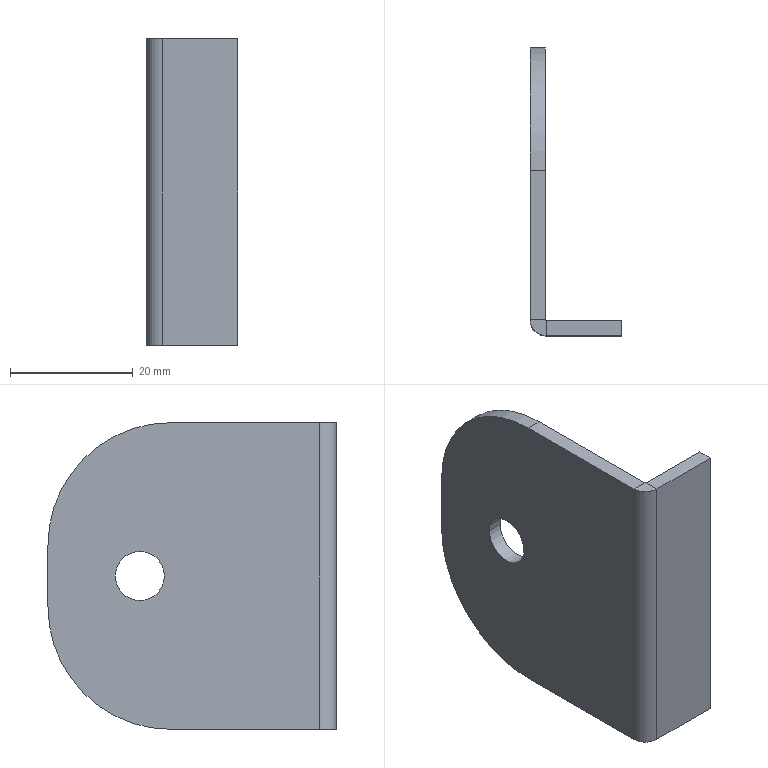Component | SolidWorks | FrontDoorAssembly-1_FrontDoorWelding-1_GasSpringSupportPG50-02-104-1 | 1 solid | 18 faces | box 15 x 47 x 50 mm | volume 6808 mm3 | plane 12 | cylinder 6 | commonest cylinder face diameters 8 x2 40 x2 5.3 x1 0.3 x1 | material AISI 1045 Steel, cold drawn
STEP:
#1=COLOUR_RGB('',0.7922,0.8196,0.9333);
#2=FILL_AREA_STYLE_COLOUR('',#1);
#3=FILL_AREA_STYLE('',(#2));
#4=SURFACE_STYLE_FILL_AREA(#3);
#5=SURFACE_SIDE_STYLE('',(#4));
#6=SURFACE_STYLE_USAGE(.BOTH.,#5);
#7=PRESENTATION_STYLE_ASSIGNMENT((#6));
#8=CARTESIAN_POINT('',(34.914,-9.992,-0.3876));
#9=VERTEX_POINT('',#8);
#10=CARTESIAN_POINT('',(34.914,-9.677,-0.3876));
#11=VERTEX_POINT('',#10);
#12=CARTESIAN_POINT('',(34.914,-9.835,-0.3876));
#13=DIRECTION('',(-1.,-0.,0.));
#14=DIRECTION('',(0.,1.,0.));
#15=AXIS2_PLACEMENT_3D('',#12,#13,#14);
#16=CIRCLE('',#15,0.1575);
#17=EDGE_CURVE('',#9,#11,#16,.T.);
#18=ORIENTED_EDGE('',*,*,#17,.F.);
#19=CARTESIAN_POINT('',(34.816,-9.992,-0.3876));
#20=VERTEX_POINT('',#19);
#21=CARTESIAN_POINT('',(34.914,-9.992,-0.3876));
#22=DIRECTION('',(-1.,-0.,0.));
#23=VECTOR('',#22,39.37);
#24=LINE('',#21,#23);
#25=EDGE_CURVE('',#9,#20,#24,.T.);
#26=ORIENTED_EDGE('',*,*,#25,.T.);
#27=CARTESIAN_POINT('',(34.816,-9.677,-0.3876));
#28=VERTEX_POINT('',#27);
#29=CARTESIAN_POINT('',(34.816,-9.835,-0.3876));
#30=DIRECTION('',(-1.,-0.,0.));
#31=DIRECTION('',(0.,1.,0.));
#32=AXIS2_PLACEMENT_3D('',#29,#30,#31);
#33=CIRCLE('',#32,0.1575);
#34=EDGE_CURVE('',#20,#28,#33,.T.);
#35=ORIENTED_EDGE('',*,*,#34,.T.);
#36=CARTESIAN_POINT('',(34.914,-9.677,-0.3876));
#37=DIRECTION('',(-1.,-0.,0.));
#38=VECTOR('',#37,39.37);
#39=LINE('',#36,#38);
#40=EDGE_CURVE('',#11,#28,#39,.T.);
#41=ORIENTED_EDGE('',*,*,#40,.F.);
#42=EDGE_LOOP('',(#18,#26,#35,#41));
#43=FACE_OUTER_BOUND('',#42,.T.);
#44=CARTESIAN_POINT('',(34.914,-9.835,-0.3876));
#45=DIRECTION('',(-1.,-0.,0.));
#46=DIRECTION('',(0.,1.,0.));
#47=AXIS2_PLACEMENT_3D('',#44,#45,#46);
#48=CYLINDRICAL_SURFACE('',#47,0.1575);
#49=ADVANCED_FACE('',(#43),#48,.F.);
#50=CARTESIAN_POINT('',(34.914,-10.031,-1.372));
#51=VERTEX_POINT('',#50);
#52=CARTESIAN_POINT('',(34.914,-10.99,-1.372));
#53=VERTEX_POINT('',#52);
#54=CARTESIAN_POINT('',(34.914,-10.031,-1.372));
#55=DIRECTION('',(0.,-1.,-0.));
#56=VECTOR('',#55,39.37);
#57=LINE('',#54,#56);
#58=EDGE_CURVE('',#51,#53,#57,.T.);
#59=ORIENTED_EDGE('',*,*,#58,.T.);
#60=CARTESIAN_POINT('',(34.816,-10.99,-1.372));
#61=VERTEX_POINT('',#60);
#62=CARTESIAN_POINT('',(34.914,-10.99,-1.372));
#63=DIRECTION('',(-1.,-0.,0.));
#64=VECTOR('',#63,39.37);
#65=LINE('',#62,#64);
#66=EDGE_CURVE('',#53,#61,#65,.T.);
#67=ORIENTED_EDGE('',*,*,#66,.T.);
#68=CARTESIAN_POINT('',(34.816,-10.031,-1.372));
#69=VERTEX_POINT('',#68);
#70=CARTESIAN_POINT('',(34.816,-10.031,-1.372));
#71=DIRECTION('',(0.,-1.,-0.));
#72=VECTOR('',#71,39.37);
#73=LINE('',#70,#72);
#74=EDGE_CURVE('',#69,#61,#73,.T.);
#75=ORIENTED_EDGE('',*,*,#74,.F.);
#76=CARTESIAN_POINT('',(34.914,-10.031,-1.372));
#77=DIRECTION('',(-1.,-0.,0.));
#78=VECTOR('',#77,39.37);
#79=LINE('',#76,#78);
#80=EDGE_CURVE('',#51,#69,#79,.T.);
#81=ORIENTED_EDGE('',*,*,#80,.F.);
#82=EDGE_LOOP('',(#59,#67,#75,#81));
#83=FACE_OUTER_BOUND('',#82,.T.);
#84=CARTESIAN_POINT('',(34.914,-10.031,-1.372));
#85=DIRECTION('',(-0.,0.,-1.));
#86=DIRECTION('',(-1.,-0.,0.));
#87=AXIS2_PLACEMENT_3D('',#84,#85,#86);
#88=PLANE('',#87);
#89=ADVANCED_FACE('',(#83),#88,.T.);
#90=CARTESIAN_POINT('',(34.914,-9.835,-0.3876));
#91=DIRECTION('',(-1.,-0.,0.));
#92=DIRECTION('',(0.,1.,0.));
#93=AXIS2_PLACEMENT_3D('',#90,#91,#92);
#94=CIRCLE('',#93,0.1575);
#95=EDGE_CURVE('',#11,#9,#94,.T.);
#96=ORIENTED_EDGE('',*,*,#95,.T.);
#97=ORIENTED_EDGE('',*,*,#17,.T.);
#98=EDGE_LOOP('',(#96,#97));
#99=FACE_BOUND('',#98,.T.);
#100=CARTESIAN_POINT('',(34.914,-10.99,0.5966));
#101=VERTEX_POINT('',#100);
#102=CARTESIAN_POINT('',(34.914,-10.99,-1.372));
#103=DIRECTION('',(0.,-0.,1.));
#104=VECTOR('',#103,39.37);
#105=LINE('',#102,#104);
#106=EDGE_CURVE('',#53,#101,#105,.T.);
#107=ORIENTED_EDGE('',*,*,#106,.F.);
#108=ORIENTED_EDGE('',*,*,#58,.F.);
#109=CARTESIAN_POINT('',(34.914,-9.244,-0.5845));
#110=VERTEX_POINT('',#109);
#111=CARTESIAN_POINT('',(34.914,-10.031,-0.5845));
#112=DIRECTION('',(-1.,-0.,0.));
#113=DIRECTION('',(-0.,1.,0.));
#114=AXIS2_PLACEMENT_3D('',#111,#112,#113);
#115=CIRCLE('',#114,0.7874);
#116=EDGE_CURVE('',#110,#51,#115,.T.);
#117=ORIENTED_EDGE('',*,*,#116,.F.);
#118=CARTESIAN_POINT('',(34.914,-9.244,-0.1908));
#119=VERTEX_POINT('',#118);
#120=CARTESIAN_POINT('',(34.914,-9.244,-0.1908));
#121=DIRECTION('',(-0.,0.,-1.));
#122=VECTOR('',#121,39.37);
#123=LINE('',#120,#122);
#124=EDGE_CURVE('',#119,#110,#123,.T.);
#125=ORIENTED_EDGE('',*,*,#124,.F.);
#126=CARTESIAN_POINT('',(34.914,-10.031,0.5966));
#127=VERTEX_POINT('',#126);
#128=CARTESIAN_POINT('',(34.914,-10.031,-0.1908));
#129=DIRECTION('',(-1.,-0.,0.));
#130=DIRECTION('',(-0.,1.,0.));
#131=AXIS2_PLACEMENT_3D('',#128,#129,#130);
#132=CIRCLE('',#131,0.7874);
#133=EDGE_CURVE('',#127,#119,#132,.T.);
#134=ORIENTED_EDGE('',*,*,#133,.F.);
#135=CARTESIAN_POINT('',(34.914,-11.094,0.5966));
#136=DIRECTION('',(-0.,1.,0.));
#137=VECTOR('',#136,39.37);
#138=LINE('',#135,#137);
#139=EDGE_CURVE('',#101,#127,#138,.T.);
#140=ORIENTED_EDGE('',*,*,#139,.F.);
#141=EDGE_LOOP('',(#107,#108,#117,#125,#134,#140));
#142=FACE_OUTER_BOUND('',#141,.T.);
#143=CARTESIAN_POINT('',(34.914,-10.031,-0.1908));
#144=DIRECTION('',(-1.,-0.,0.));
#145=DIRECTION('',(-0.,1.,0.));
#146=AXIS2_PLACEMENT_3D('',#143,#144,#145);
#147=PLANE('',#146);
#148=ADVANCED_FACE('',(#99,#142),#147,.F.);
#149=CARTESIAN_POINT('',(34.816,-9.835,-0.3876));
#150=DIRECTION('',(-1.,-0.,0.));
#151=DIRECTION('',(0.,1.,0.));
#152=AXIS2_PLACEMENT_3D('',#149,#150,#151);
#153=CIRCLE('',#152,0.1575);
#154=EDGE_CURVE('',#28,#20,#153,.T.);
#155=ORIENTED_EDGE('',*,*,#154,.F.);
#156=ORIENTED_EDGE('',*,*,#34,.F.);
#157=EDGE_LOOP('',(#155,#156));
#158=FACE_BOUND('',#157,.T.);
#159=ORIENTED_EDGE('',*,*,#74,.T.);
#160=CARTESIAN_POINT('',(34.816,-10.99,0.5966));
#161=VERTEX_POINT('',#160);
#162=CARTESIAN_POINT('',(34.816,-10.99,-1.372));
#163=DIRECTION('',(0.,-0.,1.));
#164=VECTOR('',#163,39.37);
#165=LINE('',#162,#164);
#166=EDGE_CURVE('',#61,#161,#165,.T.);
#167=ORIENTED_EDGE('',*,*,#166,.T.);
#168=CARTESIAN_POINT('',(34.816,-10.031,0.5966));
#169=VERTEX_POINT('',#168);
#170=CARTESIAN_POINT('',(34.816,-11.094,0.5966));
#171=DIRECTION('',(-0.,1.,0.));
#172=VECTOR('',#171,39.37);
#173=LINE('',#170,#172);
#174=EDGE_CURVE('',#161,#169,#173,.T.);
#175=ORIENTED_EDGE('',*,*,#174,.T.);
#176=CARTESIAN_POINT('',(34.816,-9.244,-0.1908));
#177=VERTEX_POINT('',#176);
#178=CARTESIAN_POINT('',(34.816,-10.031,-0.1908));
#179=DIRECTION('',(-1.,-0.,0.));
#180=DIRECTION('',(-0.,1.,0.));
#181=AXIS2_PLACEMENT_3D('',#178,#179,#180);
#182=CIRCLE('',#181,0.7874);
#183=EDGE_CURVE('',#169,#177,#182,.T.);
#184=ORIENTED_EDGE('',*,*,#183,.T.);
#185=CARTESIAN_POINT('',(34.816,-9.244,-0.5845));
#186=VERTEX_POINT('',#185);
#187=CARTESIAN_POINT('',(34.816,-9.244,-0.1908));
#188=DIRECTION('',(-0.,0.,-1.));
#189=VECTOR('',#188,39.37);
#190=LINE('',#187,#189);
#191=EDGE_CURVE('',#177,#186,#190,.T.);
#192=ORIENTED_EDGE('',*,*,#191,.T.);
#193=CARTESIAN_POINT('',(34.816,-10.031,-0.5845));
#194=DIRECTION('',(-1.,-0.,0.));
#195=DIRECTION('',(-0.,1.,0.));
#196=AXIS2_PLACEMENT_3D('',#193,#194,#195);
#197=CIRCLE('',#196,0.7874);
#198=EDGE_CURVE('',#186,#69,#197,.T.);
#199=ORIENTED_EDGE('',*,*,#198,.T.);
#200=EDGE_LOOP('',(#159,#167,#175,#184,#192,#199));
#201=FACE_OUTER_BOUND('',#200,.T.);
#202=CARTESIAN_POINT('',(34.816,-10.031,-0.1908));
#203=DIRECTION('',(-1.,-0.,0.));
#204=DIRECTION('',(-0.,1.,0.));
#205=AXIS2_PLACEMENT_3D('',#202,#203,#204);
#206=PLANE('',#205);
#207=ADVANCED_FACE('',(#158,#201),#206,.T.);
#208=ORIENTED_EDGE('',*,*,#198,.F.);
#209=CARTESIAN_POINT('',(34.914,-9.244,-0.5845));
#210=DIRECTION('',(-1.,-0.,0.));
#211=VECTOR('',#210,39.37);
#212=LINE('',#209,#211);
#213=EDGE_CURVE('',#110,#186,#212,.T.);
#214=ORIENTED_EDGE('',*,*,#213,.F.);
#215=ORIENTED_EDGE('',*,*,#116,.T.);
#216=ORIENTED_EDGE('',*,*,#80,.T.);
#217=EDGE_LOOP('',(#208,#214,#215,#216));
#218=FACE_OUTER_BOUND('',#217,.T.);
#219=CARTESIAN_POINT('',(34.914,-10.031,-0.5845));
#220=DIRECTION('',(-1.,-0.,0.));
#221=DIRECTION('',(-0.,1.,0.));
#222=AXIS2_PLACEMENT_3D('',#219,#220,#221);
#223=CYLINDRICAL_SURFACE('',#222,0.7874);
#224=ADVANCED_FACE('',(#218),#223,.T.);
#225=ORIENTED_EDGE('',*,*,#191,.F.);
#226=CARTESIAN_POINT('',(34.914,-9.244,-0.1908));
#227=DIRECTION('',(-1.,-0.,0.));
#228=VECTOR('',#227,39.37);
#229=LINE('',#226,#228);
#230=EDGE_CURVE('',#119,#177,#229,.T.);
#231=ORIENTED_EDGE('',*,*,#230,.F.);
#232=ORIENTED_EDGE('',*,*,#124,.T.);
#233=ORIENTED_EDGE('',*,*,#213,.T.);
#234=EDGE_LOOP('',(#225,#231,#232,#233));
#235=FACE_OUTER_BOUND('',#234,.T.);
#236=CARTESIAN_POINT('',(34.914,-9.244,-0.1908));
#237=DIRECTION('',(-0.,1.,0.));
#238=DIRECTION('',(1.,0.,-0.));
#239=AXIS2_PLACEMENT_3D('',#236,#237,#238);
#240=PLANE('',#239);
#241=ADVANCED_FACE('',(#235),#240,.T.);
#242=ORIENTED_EDGE('',*,*,#183,.F.);
#243=CARTESIAN_POINT('',(34.914,-10.031,0.5966));
#244=DIRECTION('',(-1.,-0.,0.));
#245=VECTOR('',#244,39.37);
#246=LINE('',#243,#245);
#247=EDGE_CURVE('',#127,#169,#246,.T.);
#248=ORIENTED_EDGE('',*,*,#247,.F.);
#249=ORIENTED_EDGE('',*,*,#133,.T.);
#250=ORIENTED_EDGE('',*,*,#230,.T.);
#251=EDGE_LOOP('',(#242,#248,#249,#250));
#252=FACE_OUTER_BOUND('',#251,.T.);
#253=CARTESIAN_POINT('',(34.914,-10.031,-0.1908));
#254=DIRECTION('',(-1.,-0.,0.));
#255=DIRECTION('',(-0.,1.,0.));
#256=AXIS2_PLACEMENT_3D('',#253,#254,#255);
#257=CYLINDRICAL_SURFACE('',#256,0.7874);
#258=ADVANCED_FACE('',(#252),#257,.T.);
#259=CARTESIAN_POINT('',(34.914,-10.99,0.5966));
#260=DIRECTION('',(-1.,-0.,0.));
#261=VECTOR('',#260,39.37);
#262=LINE('',#259,#261);
#263=EDGE_CURVE('',#101,#161,#262,.T.);
#264=ORIENTED_EDGE('',*,*,#263,.F.);
#265=ORIENTED_EDGE('',*,*,#139,.T.);
#266=ORIENTED_EDGE('',*,*,#247,.T.);
#267=ORIENTED_EDGE('',*,*,#174,.F.);
#268=EDGE_LOOP('',(#264,#265,#266,#267));
#269=FACE_OUTER_BOUND('',#268,.T.);
#270=CARTESIAN_POINT('',(34.914,-11.094,0.5966));
#271=DIRECTION('',(0.,-0.,1.));
#272=DIRECTION('',(1.,0.,-0.));
#273=AXIS2_PLACEMENT_3D('',#270,#271,#272);
#274=PLANE('',#273);
#275=ADVANCED_FACE('',(#269),#274,.T.);
#276=ORIENTED_EDGE('',*,*,#25,.F.);
#277=ORIENTED_EDGE('',*,*,#95,.F.);
#278=ORIENTED_EDGE('',*,*,#40,.T.);
#279=ORIENTED_EDGE('',*,*,#154,.T.);
#280=EDGE_LOOP('',(#276,#277,#278,#279));
#281=FACE_OUTER_BOUND('',#280,.T.);
#282=CARTESIAN_POINT('',(34.914,-9.835,-0.3876));
#283=DIRECTION('',(-1.,-0.,0.));
#284=DIRECTION('',(0.,1.,0.));
#285=AXIS2_PLACEMENT_3D('',#282,#283,#284);
#286=CYLINDRICAL_SURFACE('',#285,0.1575);
#287=ADVANCED_FACE('',(#281),#286,.F.);
#288=CARTESIAN_POINT('',(34.92,-10.996,0.5966));
#289=VERTEX_POINT('',#288);
#290=CARTESIAN_POINT('',(34.92,-11.094,0.5966));
#291=VERTEX_POINT('',#290);
#292=CARTESIAN_POINT('',(34.92,-11.094,0.5966));
#293=DIRECTION('',(0.,-1.,-0.));
#294=VECTOR('',#293,39.37);
#295=LINE('',#292,#294);
#296=EDGE_CURVE('',#289,#291,#295,.T.);
#297=ORIENTED_EDGE('',*,*,#296,.F.);
#298=CARTESIAN_POINT('',(34.92,-10.99,0.5966));
#299=DIRECTION('',(0.,-0.,1.));
#300=DIRECTION('',(-1.,0.,0.));
#301=AXIS2_PLACEMENT_3D('',#298,#299,#300);
#302=CIRCLE('',#301,0.005906);
#303=EDGE_CURVE('',#101,#289,#302,.T.);
#304=ORIENTED_EDGE('',*,*,#303,.F.);
#305=ORIENTED_EDGE('',*,*,#263,.T.);
#306=CARTESIAN_POINT('',(34.92,-10.99,0.5966));
#307=DIRECTION('',(0.,-0.,1.));
#308=DIRECTION('',(-1.,0.,0.));
#309=AXIS2_PLACEMENT_3D('',#306,#307,#308);
#310=CIRCLE('',#309,0.1043);
#311=EDGE_CURVE('',#161,#291,#310,.T.);
#312=ORIENTED_EDGE('',*,*,#311,.T.);
#313=EDGE_LOOP('',(#297,#304,#305,#312));
#314=FACE_OUTER_BOUND('',#313,.T.);
#315=CARTESIAN_POINT('',(34.92,-10.99,0.5966));
#316=DIRECTION('',(0.,-0.,1.));
#317=DIRECTION('',(1.,0.,-0.));
#318=AXIS2_PLACEMENT_3D('',#315,#316,#317);
#319=PLANE('',#318);
#320=ADVANCED_FACE('',(#314),#319,.T.);
#321=CARTESIAN_POINT('',(34.92,-10.996,-1.372));
#322=VERTEX_POINT('',#321);
#323=CARTESIAN_POINT('',(34.92,-10.99,-1.372));
#324=DIRECTION('',(-0.,0.,-1.));
#325=DIRECTION('',(-1.,0.,0.));
#326=AXIS2_PLACEMENT_3D('',#323,#324,#325);
#327=CIRCLE('',#326,0.005906);
#328=EDGE_CURVE('',#322,#53,#327,.T.);
#329=ORIENTED_EDGE('',*,*,#328,.F.);
#330=CARTESIAN_POINT('',(34.92,-11.094,-1.372));
#331=VERTEX_POINT('',#330);
#332=CARTESIAN_POINT('',(34.92,-10.996,-1.372));
#333=DIRECTION('',(0.,-1.,-0.));
#334=VECTOR('',#333,39.37);
#335=LINE('',#332,#334);
#336=EDGE_CURVE('',#322,#331,#335,.T.);
#337=ORIENTED_EDGE('',*,*,#336,.T.);
#338=CARTESIAN_POINT('',(34.92,-10.99,-1.372));
#339=DIRECTION('',(-0.,0.,-1.));
#340=DIRECTION('',(-1.,0.,0.));
#341=AXIS2_PLACEMENT_3D('',#338,#339,#340);
#342=CIRCLE('',#341,0.1043);
#343=EDGE_CURVE('',#331,#61,#342,.T.);
#344=ORIENTED_EDGE('',*,*,#343,.T.);
#345=ORIENTED_EDGE('',*,*,#66,.F.);
#346=EDGE_LOOP('',(#329,#337,#344,#345));
#347=FACE_OUTER_BOUND('',#346,.T.);
#348=CARTESIAN_POINT('',(34.92,-10.99,-1.372));
#349=DIRECTION('',(0.,-0.,1.));
#350=DIRECTION('',(1.,0.,-0.));
#351=AXIS2_PLACEMENT_3D('',#348,#349,#350);
#352=PLANE('',#351);
#353=ADVANCED_FACE('',(#347),#352,.F.);
#354=ORIENTED_EDGE('',*,*,#166,.F.);
#355=ORIENTED_EDGE('',*,*,#343,.F.);
#356=CARTESIAN_POINT('',(34.92,-11.094,0.5966));
#357=DIRECTION('',(0.,-0.,1.));
#358=VECTOR('',#357,39.37);
#359=LINE('',#356,#358);
#360=EDGE_CURVE('',#331,#291,#359,.T.);
#361=ORIENTED_EDGE('',*,*,#360,.T.);
#362=ORIENTED_EDGE('',*,*,#311,.F.);
#363=EDGE_LOOP('',(#354,#355,#361,#362));
#364=FACE_OUTER_BOUND('',#363,.T.);
#365=CARTESIAN_POINT('',(34.92,-10.99,-1.372));
#366=DIRECTION('',(-0.,0.,-1.));
#367=DIRECTION('',(0.,-1.,0.));
#368=AXIS2_PLACEMENT_3D('',#365,#366,#367);
#369=CYLINDRICAL_SURFACE('',#368,0.1043);
#370=ADVANCED_FACE('',(#364),#369,.T.);
#371=ORIENTED_EDGE('',*,*,#106,.T.);
#372=ORIENTED_EDGE('',*,*,#303,.T.);
#373=CARTESIAN_POINT('',(34.92,-10.996,0.5966));
#374=DIRECTION('',(-0.,0.,-1.));
#375=VECTOR('',#374,39.37);
#376=LINE('',#373,#375);
#377=EDGE_CURVE('',#289,#322,#376,.T.);
#378=ORIENTED_EDGE('',*,*,#377,.T.);
#379=ORIENTED_EDGE('',*,*,#328,.T.);
#380=EDGE_LOOP('',(#371,#372,#378,#379));
#381=FACE_OUTER_BOUND('',#380,.T.);
#382=CARTESIAN_POINT('',(34.92,-10.99,-1.372));
#383=DIRECTION('',(-0.,0.,-1.));
#384=DIRECTION('',(0.,-1.,0.));
#385=AXIS2_PLACEMENT_3D('',#382,#383,#384);
#386=CYLINDRICAL_SURFACE('',#385,0.005906);
#387=ADVANCED_FACE('',(#381),#386,.F.);
#388=ORIENTED_EDGE('',*,*,#336,.F.);
#389=CARTESIAN_POINT('',(35.406,-10.996,-1.372));
#390=VERTEX_POINT('',#389);
#391=CARTESIAN_POINT('',(35.406,-10.996,-1.372));
#392=DIRECTION('',(1.,0.,-0.));
#393=VECTOR('',#392,39.37);
#394=LINE('',#391,#393);
#395=EDGE_CURVE('',#322,#390,#394,.T.);
#396=ORIENTED_EDGE('',*,*,#395,.T.);
#397=CARTESIAN_POINT('',(35.406,-11.094,-1.372));
#398=VERTEX_POINT('',#397);
#399=CARTESIAN_POINT('',(35.406,-11.094,-1.372));
#400=DIRECTION('',(-0.,1.,0.));
#401=VECTOR('',#400,39.37);
#402=LINE('',#399,#401);
#403=EDGE_CURVE('',#398,#390,#402,.T.);
#404=ORIENTED_EDGE('',*,*,#403,.F.);
#405=CARTESIAN_POINT('',(34.816,-11.094,-1.372));
#406=DIRECTION('',(1.,0.,-0.));
#407=VECTOR('',#406,39.37);
#408=LINE('',#405,#407);
#409=EDGE_CURVE('',#331,#398,#408,.T.);
#410=ORIENTED_EDGE('',*,*,#409,.F.);
#411=EDGE_LOOP('',(#388,#396,#404,#410));
#412=FACE_OUTER_BOUND('',#411,.T.);
#413=CARTESIAN_POINT('',(35.406,-11.094,-1.372));
#414=DIRECTION('',(0.,-0.,1.));
#415=DIRECTION('',(1.,0.,-0.));
#416=AXIS2_PLACEMENT_3D('',#413,#414,#415);
#417=PLANE('',#416);
#418=ADVANCED_FACE('',(#412),#417,.F.);
#419=ORIENTED_EDGE('',*,*,#296,.T.);
#420=CARTESIAN_POINT('',(35.406,-11.094,0.5966));
#421=VERTEX_POINT('',#420);
#422=CARTESIAN_POINT('',(34.816,-11.094,0.5966));
#423=DIRECTION('',(-1.,-0.,0.));
#424=VECTOR('',#423,39.37);
#425=LINE('',#422,#424);
#426=EDGE_CURVE('',#421,#291,#425,.T.);
#427=ORIENTED_EDGE('',*,*,#426,.F.);
#428=CARTESIAN_POINT('',(35.406,-10.996,0.5966));
#429=VERTEX_POINT('',#428);
#430=CARTESIAN_POINT('',(35.406,-11.094,0.5966));
#431=DIRECTION('',(-0.,1.,0.));
#432=VECTOR('',#431,39.37);
#433=LINE('',#430,#432);
#434=EDGE_CURVE('',#421,#429,#433,.T.);
#435=ORIENTED_EDGE('',*,*,#434,.T.);
#436=CARTESIAN_POINT('',(34.914,-10.996,0.5966));
#437=DIRECTION('',(-1.,-0.,0.));
#438=VECTOR('',#437,39.37);
#439=LINE('',#436,#438);
#440=EDGE_CURVE('',#429,#289,#439,.T.);
#441=ORIENTED_EDGE('',*,*,#440,.T.);
#442=EDGE_LOOP('',(#419,#427,#435,#441));
#443=FACE_OUTER_BOUND('',#442,.T.);
#444=CARTESIAN_POINT('',(34.914,-11.094,0.5966));
#445=DIRECTION('',(-0.,0.,-1.));
#446=DIRECTION('',(-1.,-0.,0.));
#447=AXIS2_PLACEMENT_3D('',#444,#445,#446);
#448=PLANE('',#447);
#449=ADVANCED_FACE('',(#443),#448,.F.);
#450=ORIENTED_EDGE('',*,*,#360,.F.);
#451=ORIENTED_EDGE('',*,*,#409,.T.);
#452=CARTESIAN_POINT('',(35.406,-11.094,-0.3876));
#453=DIRECTION('',(0.,-0.,1.));
#454=VECTOR('',#453,39.37);
#455=LINE('',#452,#454);
#456=EDGE_CURVE('',#398,#421,#455,.T.);
#457=ORIENTED_EDGE('',*,*,#456,.T.);
#458=ORIENTED_EDGE('',*,*,#426,.T.);
#459=EDGE_LOOP('',(#450,#451,#457,#458));
#460=FACE_OUTER_BOUND('',#459,.T.);
#461=CARTESIAN_POINT('',(34.816,-11.094,-0.3876));
#462=DIRECTION('',(-0.,1.,0.));
#463=DIRECTION('',(1.,0.,-0.));
#464=AXIS2_PLACEMENT_3D('',#461,#462,#463);
#465=PLANE('',#464);
#466=ADVANCED_FACE('',(#460),#465,.F.);
#467=ORIENTED_EDGE('',*,*,#395,.F.);
#468=ORIENTED_EDGE('',*,*,#377,.F.);
#469=ORIENTED_EDGE('',*,*,#440,.F.);
#470=CARTESIAN_POINT('',(35.406,-10.996,0.5966));
#471=DIRECTION('',(0.,-0.,1.));
#472=VECTOR('',#471,39.37);
#473=LINE('',#470,#472);
#474=EDGE_CURVE('',#390,#429,#473,.T.);
#475=ORIENTED_EDGE('',*,*,#474,.F.);
#476=EDGE_LOOP('',(#467,#468,#469,#475));
#477=FACE_OUTER_BOUND('',#476,.T.);
#478=CARTESIAN_POINT('',(34.816,-10.996,-0.3876));
#479=DIRECTION('',(-0.,1.,0.));
#480=DIRECTION('',(1.,0.,-0.));
#481=AXIS2_PLACEMENT_3D('',#478,#479,#480);
#482=PLANE('',#481);
#483=ADVANCED_FACE('',(#477),#482,.T.);
#484=ORIENTED_EDGE('',*,*,#474,.T.);
#485=ORIENTED_EDGE('',*,*,#434,.F.);
#486=ORIENTED_EDGE('',*,*,#456,.F.);
#487=ORIENTED_EDGE('',*,*,#403,.T.);
#488=EDGE_LOOP('',(#484,#485,#486,#487));
#489=FACE_OUTER_BOUND('',#488,.T.);
#490=CARTESIAN_POINT('',(35.406,-11.094,0.5966));
#491=DIRECTION('',(-1.,-0.,0.));
#492=DIRECTION('',(-0.,1.,0.));
#493=AXIS2_PLACEMENT_3D('',#490,#491,#492);
#494=PLANE('',#493);
#495=ADVANCED_FACE('',(#489),#494,.F.);
#496=CLOSED_SHELL('',(#49,#89,#148,#207,#224,#241,#258,#275,#287,#320,#353,#370,#387,#418,#449,#466,#483,#495));
#497=MANIFOLD_SOLID_BREP('',#496);
#498=STYLED_ITEM('',(#7),#497);
#499=(LENGTH_UNIT()NAMED_UNIT(*)SI_UNIT($,.METRE.));
#500=LENGTH_MEASURE_WITH_UNIT(LENGTH_MEASURE(0.0254),#499);
#501=DIMENSIONAL_EXPONENTS(1.,0.,0.,0.,0.,0.,0.);
#502=(CONVERSION_BASED_UNIT('',#500)LENGTH_UNIT()NAMED_UNIT(#501));
#503=UNCERTAINTY_MEASURE_WITH_UNIT(LENGTH_MEASURE(0.00001),#502,'','');
#504=(NAMED_UNIT(*)PLANE_ANGLE_UNIT()SI_UNIT($,.RADIAN.));
#505=(NAMED_UNIT(*)SI_UNIT($,.STERADIAN.)SOLID_ANGLE_UNIT());
#506=(GEOMETRIC_REPRESENTATION_CONTEXT(3)GLOBAL_UNCERTAINTY_ASSIGNED_CONTEXT((#503))GLOBAL_UNIT_ASSIGNED_CONTEXT((#502,#504,#505))REPRESENTATION_CONTEXT('',''));
#507=MECHANICAL_DESIGN_GEOMETRIC_PRESENTATION_REPRESENTATION('',(#498),#506);
#508=CARTESIAN_POINT('',(0.,0.,0.));
#509=DIRECTION('',(0.,0.,1.));
#510=DIRECTION('',(1.,0.,0.));
#511=AXIS2_PLACEMENT_3D('',#508,#509,#510);
#512=(LENGTH_UNIT()NAMED_UNIT(*)SI_UNIT($,.METRE.));
#513=LENGTH_MEASURE_WITH_UNIT(LENGTH_MEASURE(0.0254),#512);
#514=DIMENSIONAL_EXPONENTS(1.,0.,0.,0.,0.,0.,0.);
#515=(CONVERSION_BASED_UNIT('',#513)LENGTH_UNIT()NAMED_UNIT(#514));
#516=UNCERTAINTY_MEASURE_WITH_UNIT(LENGTH_MEASURE(0.00001),#515,'','');
#517=(NAMED_UNIT(*)PLANE_ANGLE_UNIT()SI_UNIT($,.RADIAN.));
#518=(NAMED_UNIT(*)SI_UNIT($,.STERADIAN.)SOLID_ANGLE_UNIT());
#519=(GEOMETRIC_REPRESENTATION_CONTEXT(3)GLOBAL_UNCERTAINTY_ASSIGNED_CONTEXT((#516))GLOBAL_UNIT_ASSIGNED_CONTEXT((#515,#517,#518))REPRESENTATION_CONTEXT('',''));
#520=ADVANCED_BREP_SHAPE_REPRESENTATION('',(#497,#511),#519);
#521=PRESENTATION_LAYER_ASSIGNMENT('','',(#498));